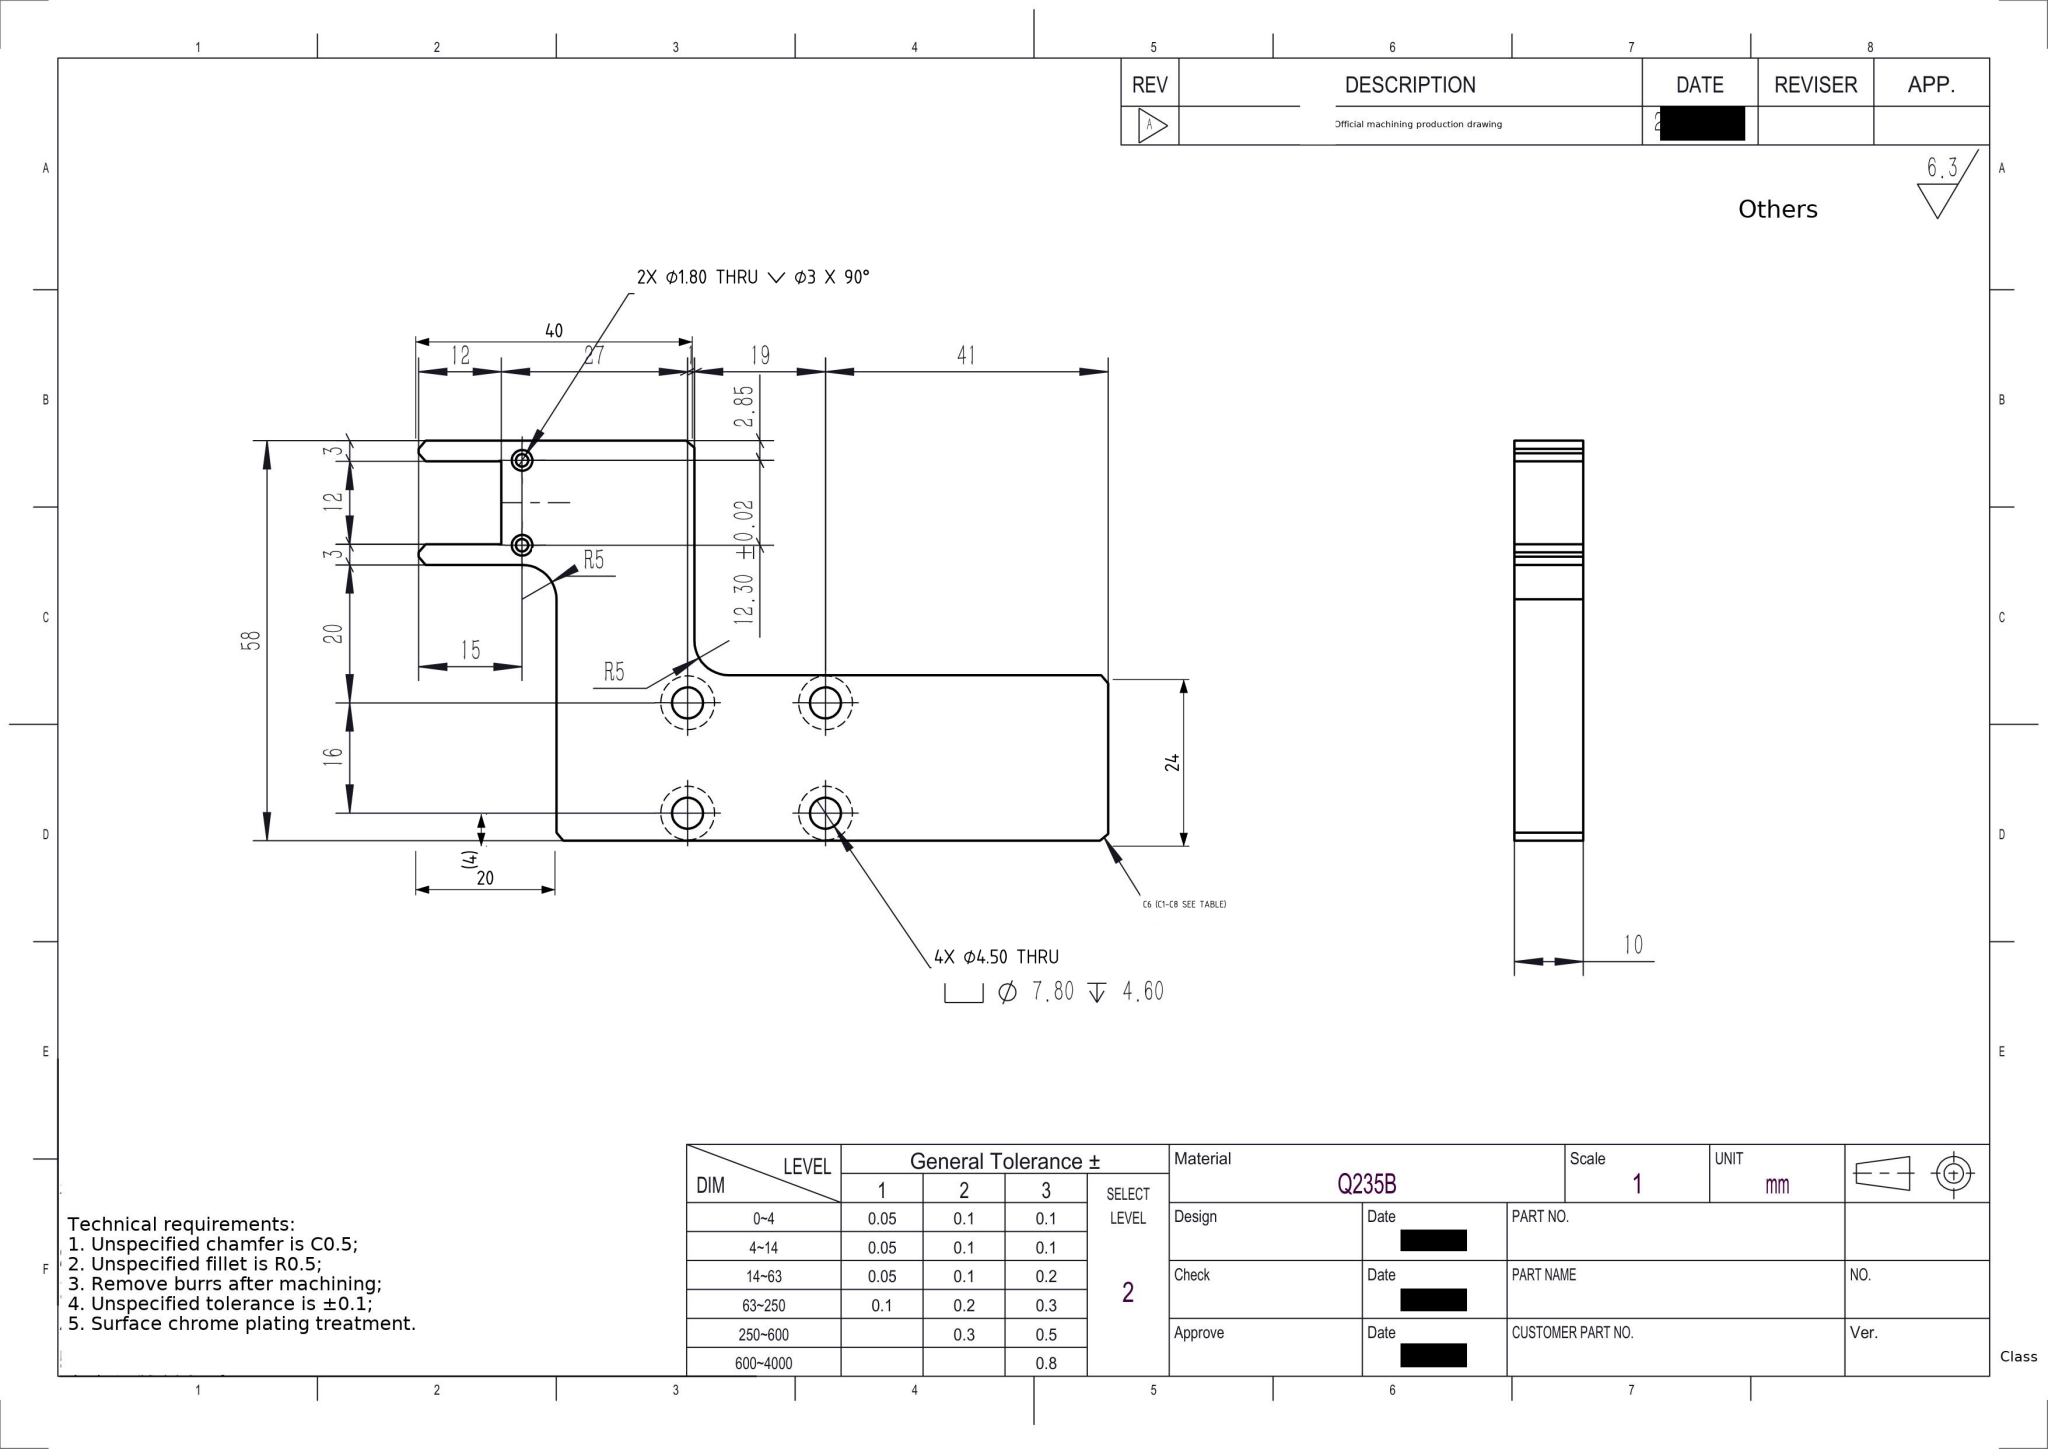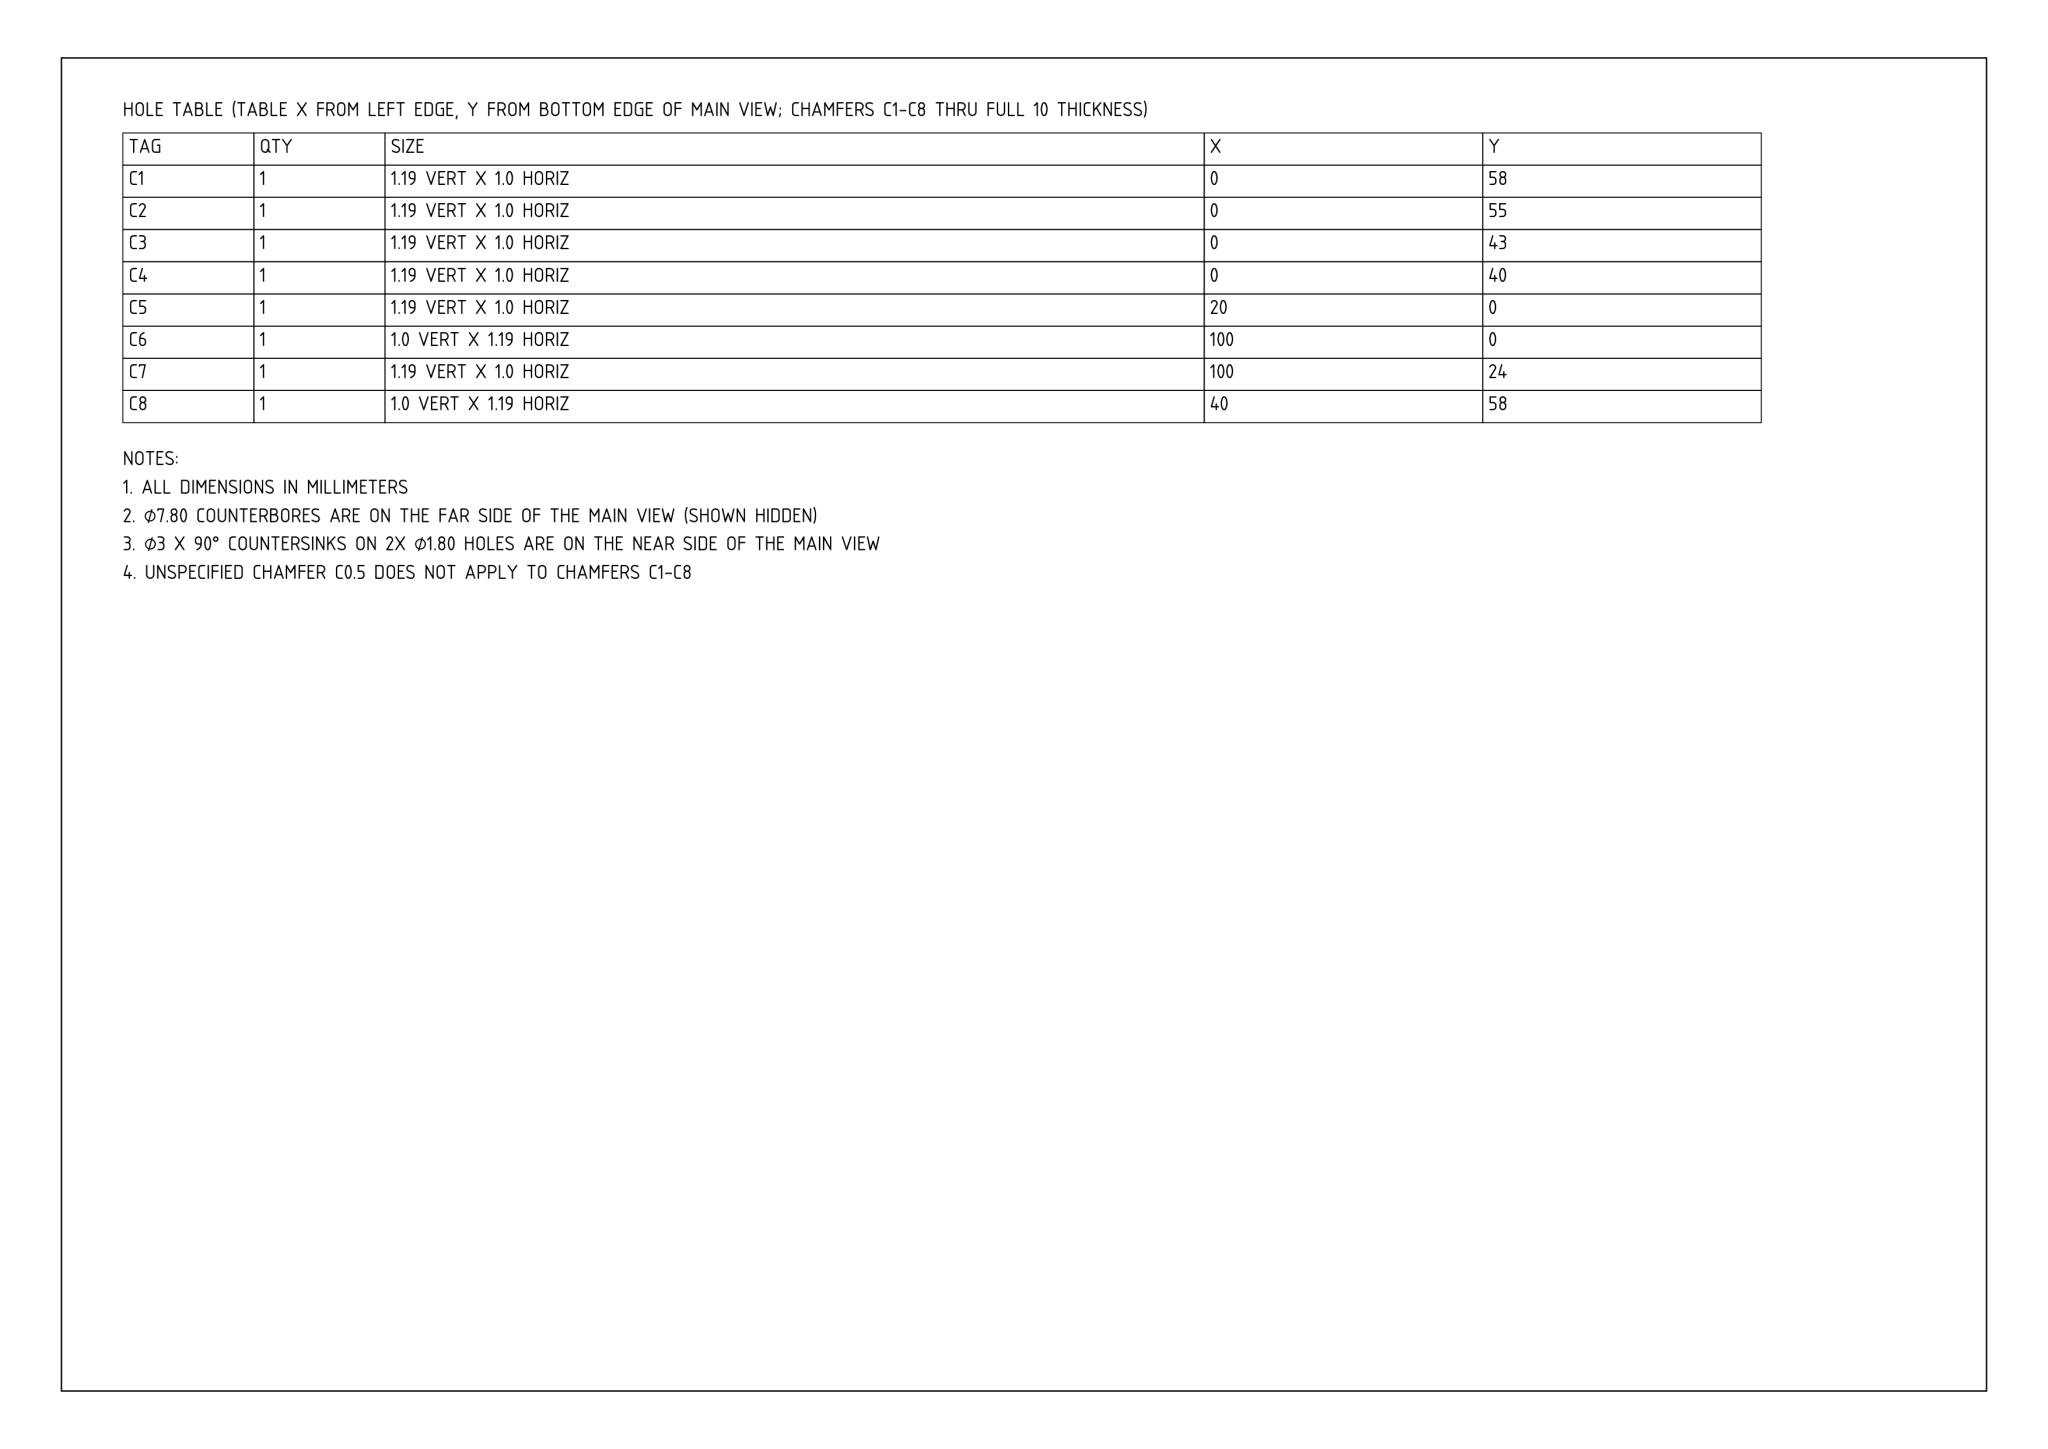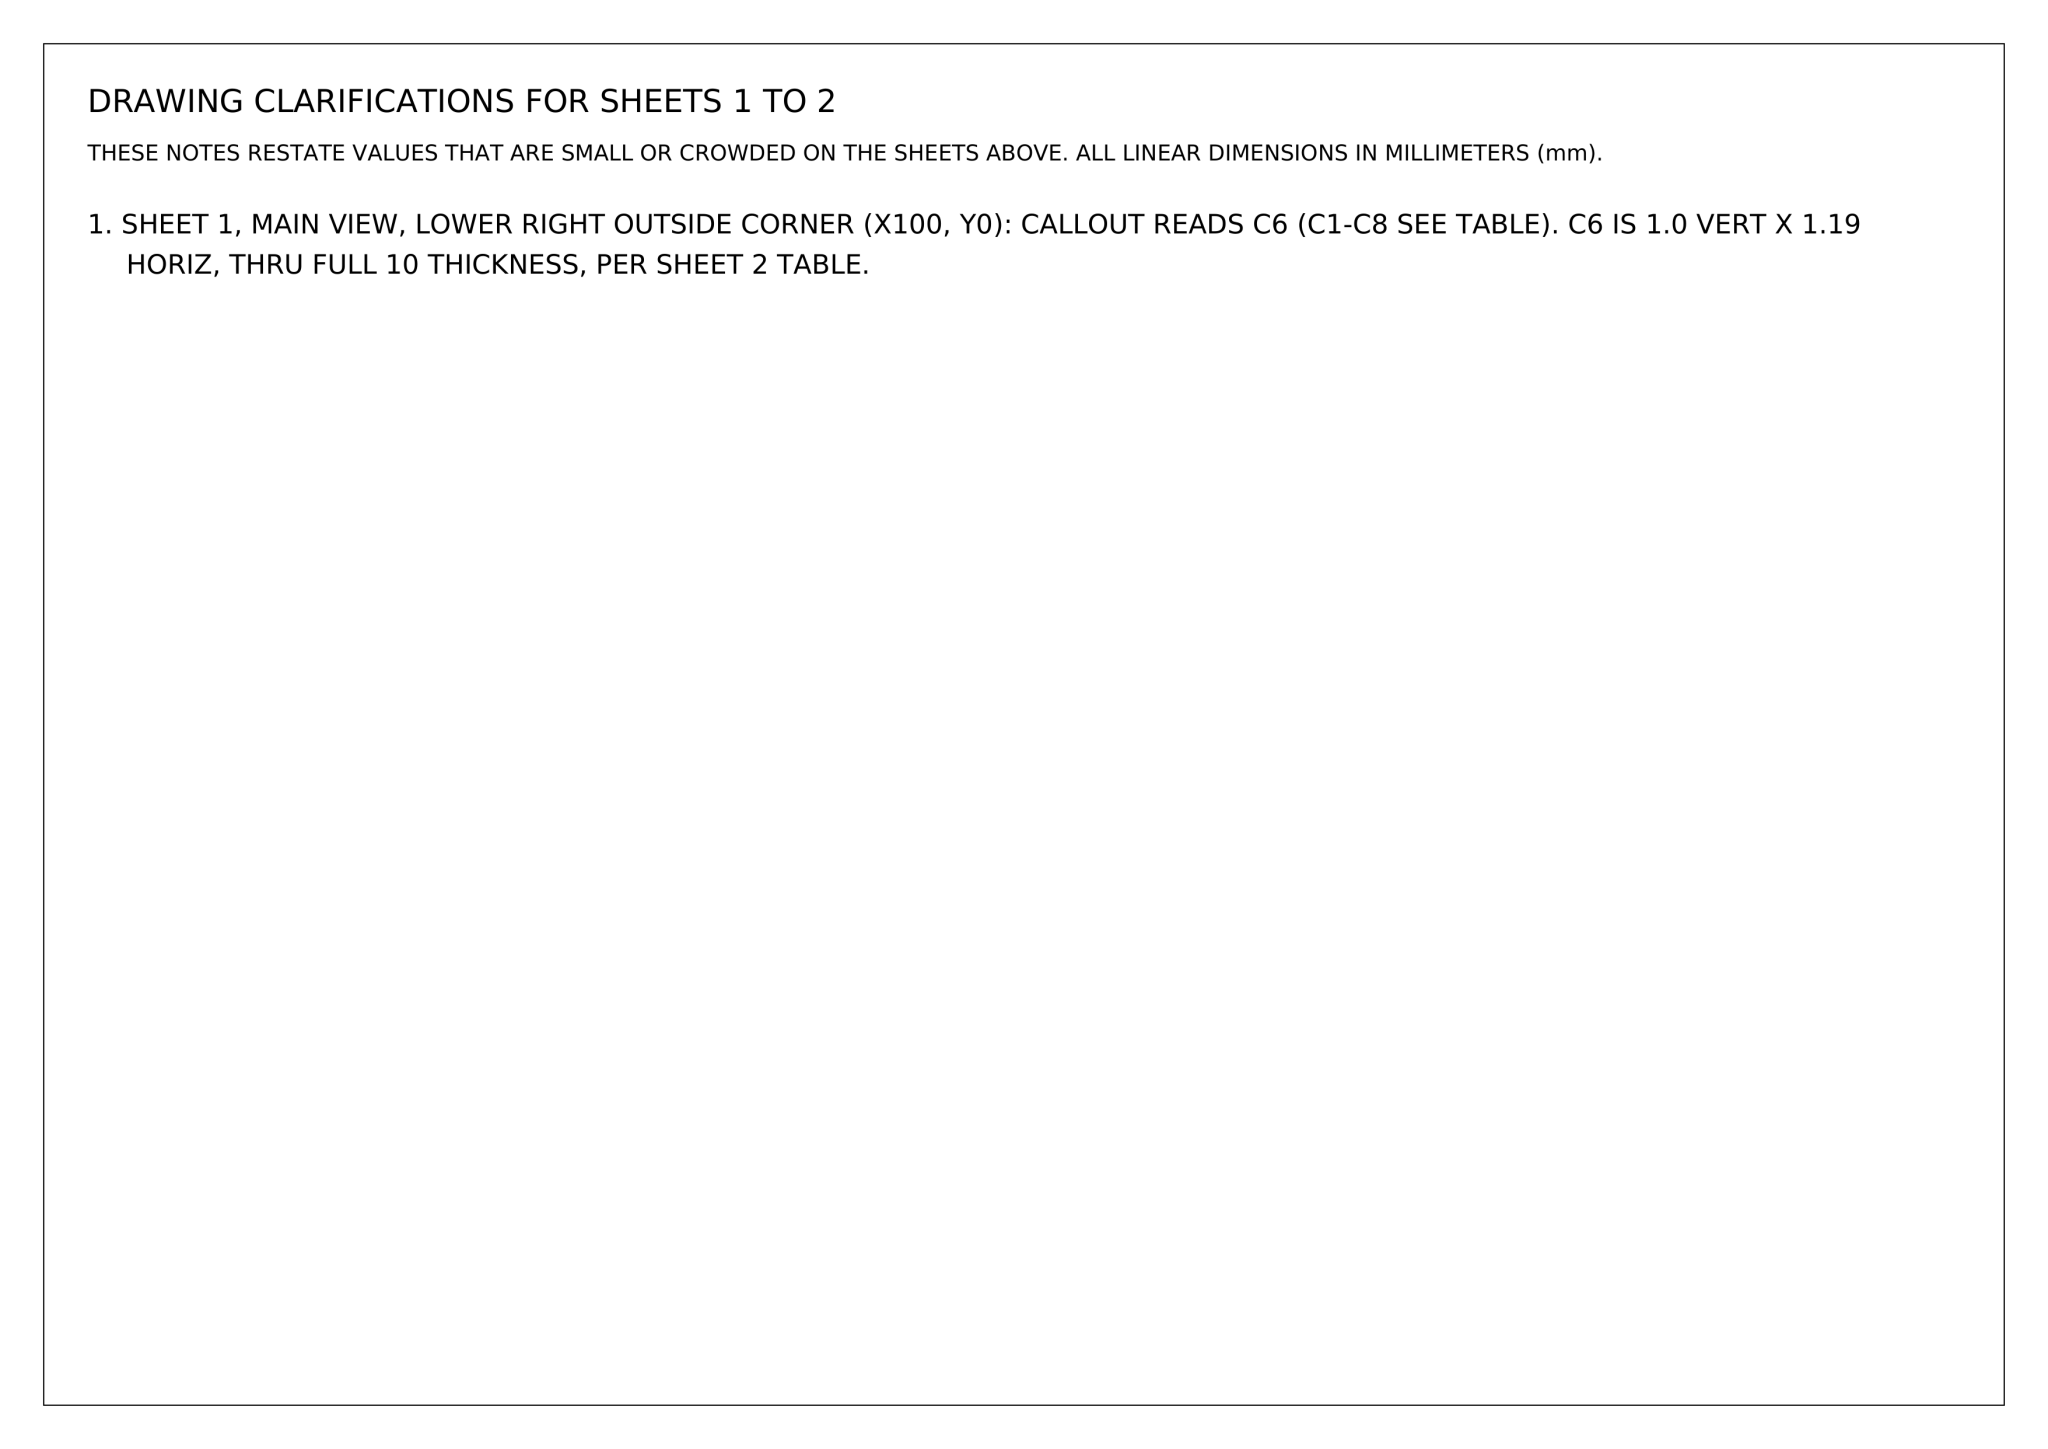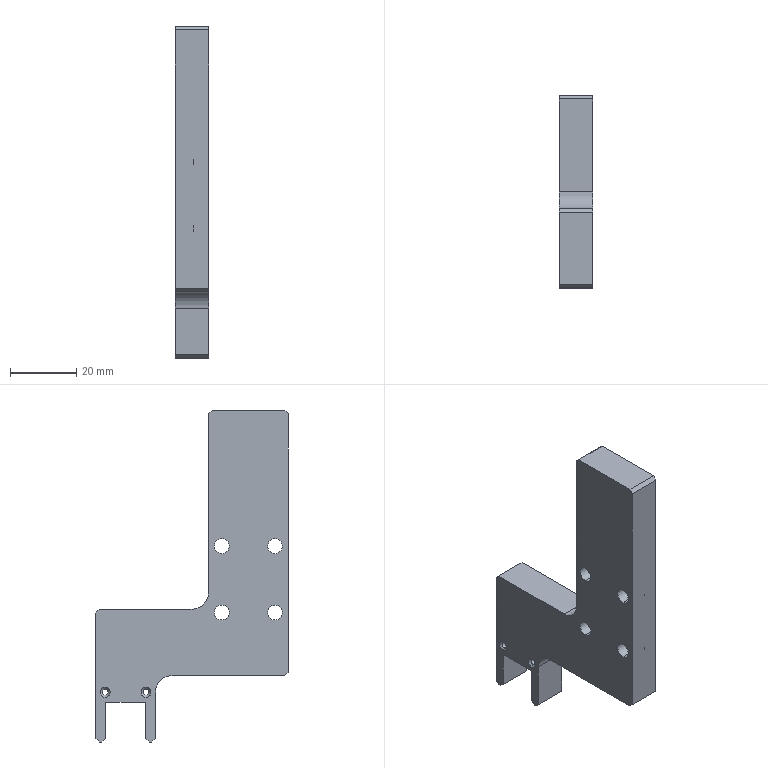Part | NX | mm | 1 solid | 52 faces | box 10 x 58 x 100 mm | volume 26943 mm3 | plane 26 | cylinder 22 | cone 4 | commonest cylinder face diameters 7.8 x8 4.5 x8 1.8 x4 10 x2